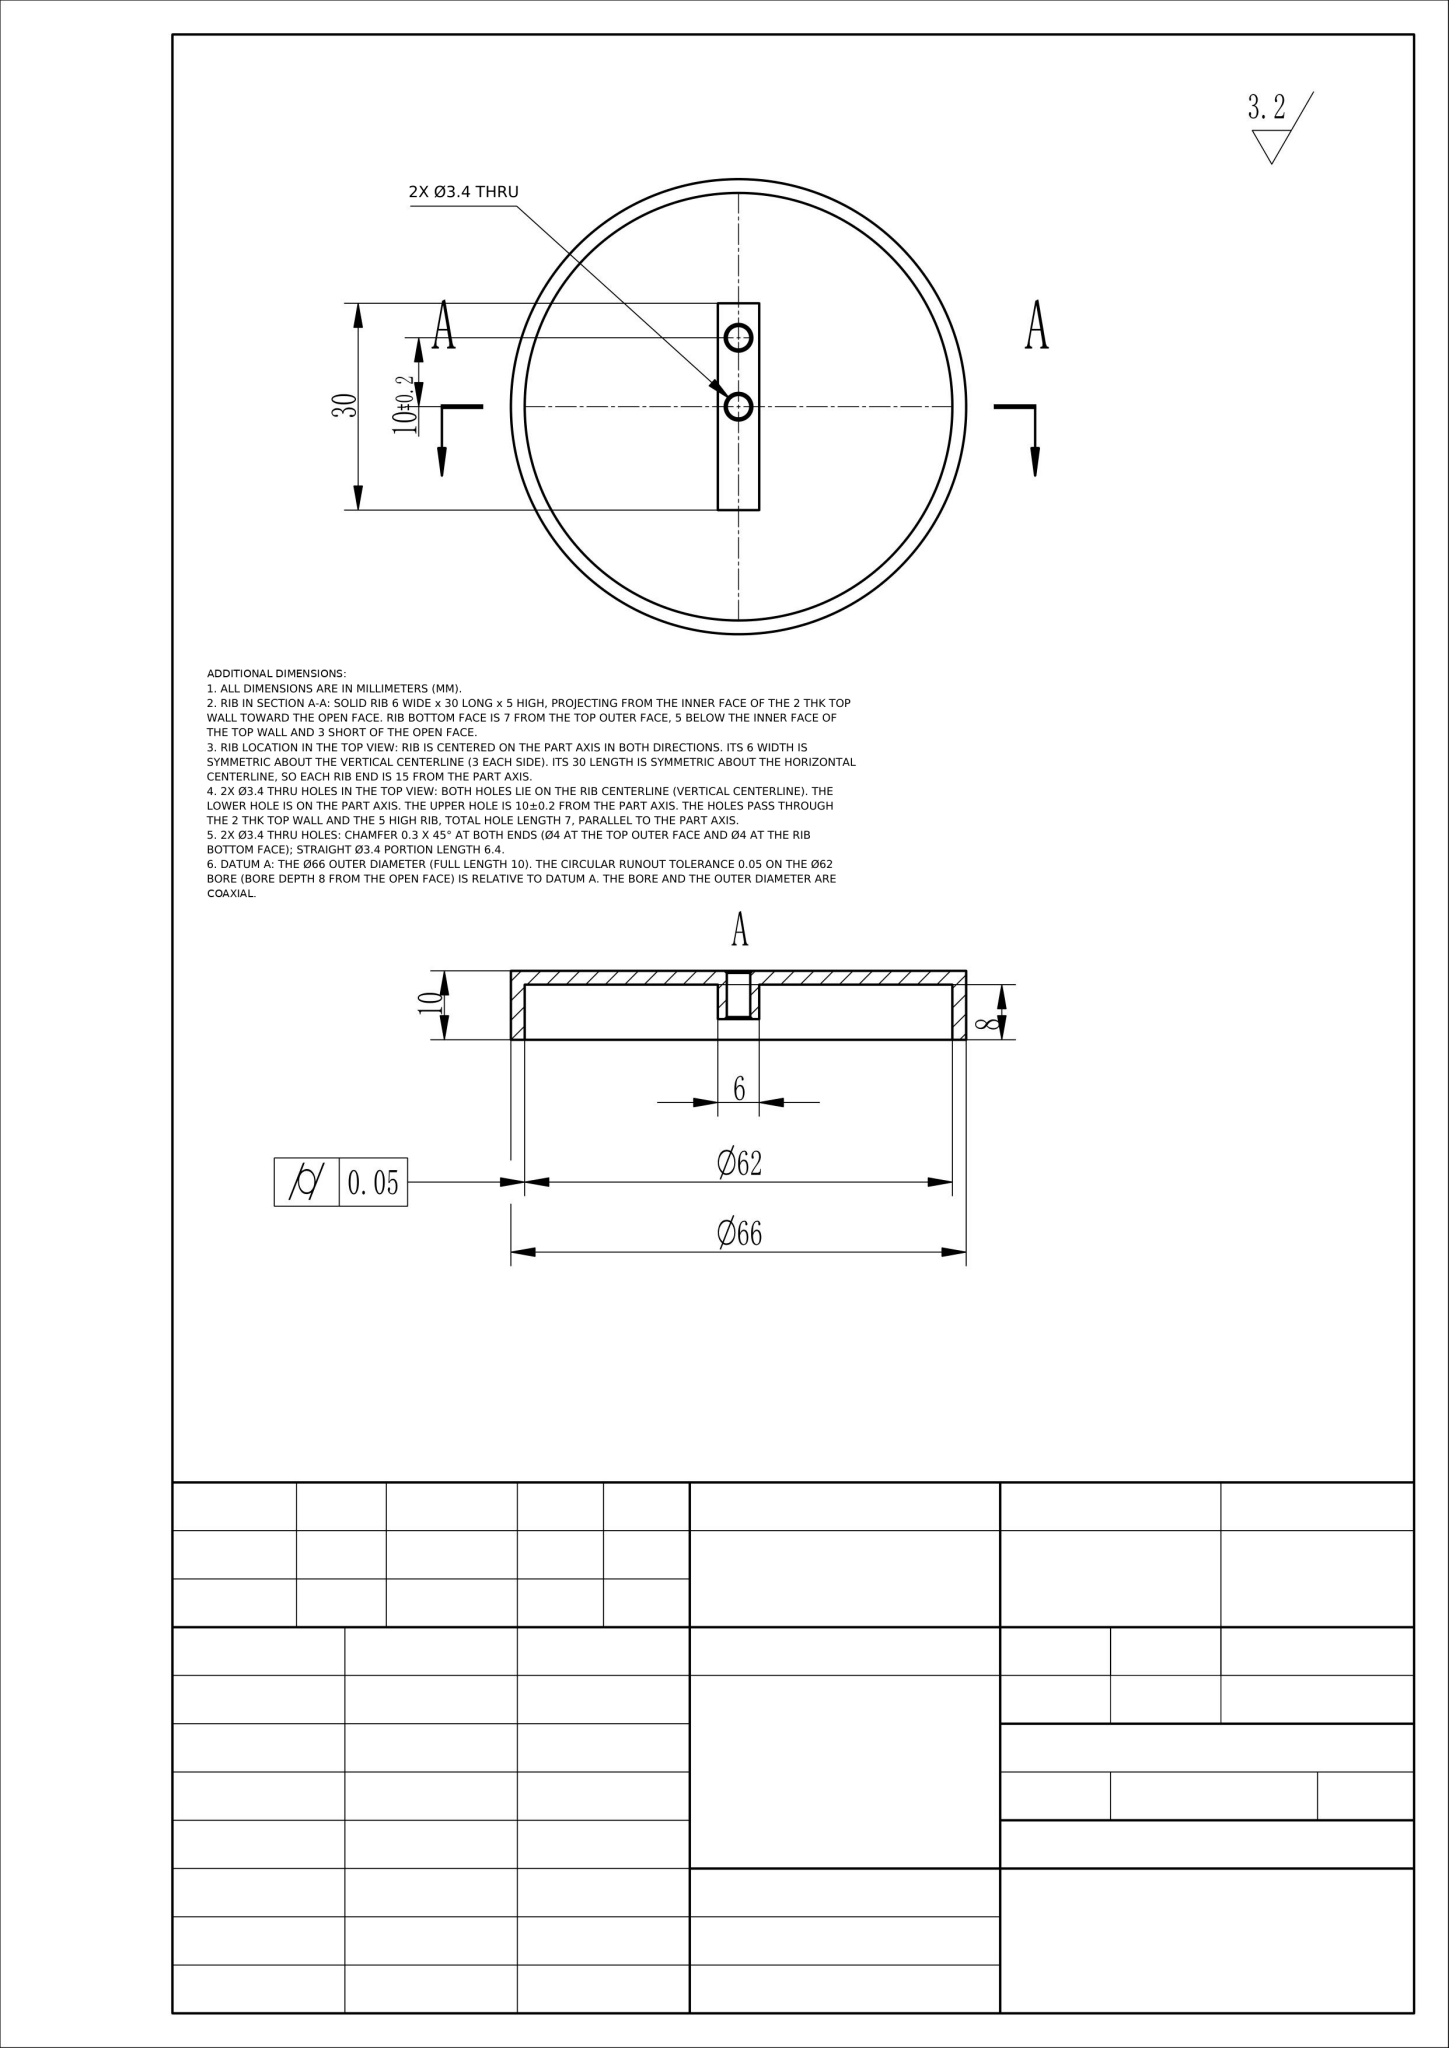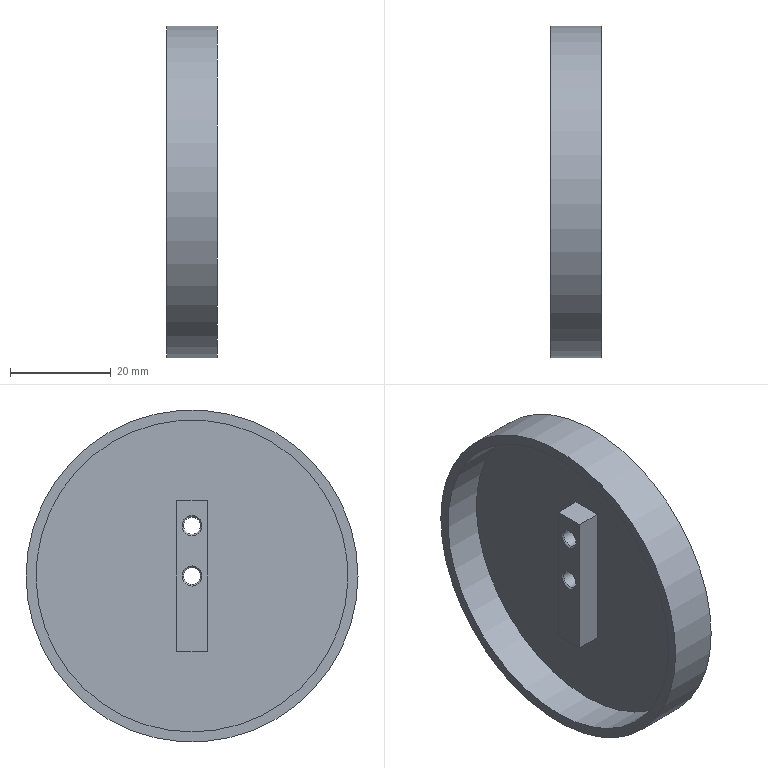Part | NX | mm | 1 solid | 16 faces | box 10 x 66 x 66 mm | volume 10830 mm3 | plane 8 | cylinder 4 | cone 4 | commonest cylinder face diameters 3.4 x2 62 x1 66 x1
STEP:
#1=CARTESIAN_POINT('',(0.,0.,0.));
#2=DIRECTION('',(0.,0.,1.));
#3=DIRECTION('',(1.,0.,0.));
#4=AXIS2_PLACEMENT_3D('',#1,#2,#3);
#5=(LENGTH_UNIT()NAMED_UNIT(*)SI_UNIT(.MILLI.,.METRE.));
#6=UNCERTAINTY_MEASURE_WITH_UNIT(LENGTH_MEASURE(0.00002),#5,'','');
#7=(NAMED_UNIT(*)PLANE_ANGLE_UNIT()SI_UNIT($,.RADIAN.));
#8=PLANE_ANGLE_MEASURE_WITH_UNIT(PLANE_ANGLE_MEASURE(0.01745),#7);
#9=DIMENSIONAL_EXPONENTS(0.,0.,0.,0.,0.,0.,0.);
#10=(CONVERSION_BASED_UNIT('',#8)NAMED_UNIT(#9)PLANE_ANGLE_UNIT());
#11=(NAMED_UNIT(*)SI_UNIT($,.STERADIAN.)SOLID_ANGLE_UNIT());
#12=(GEOMETRIC_REPRESENTATION_CONTEXT(3)GLOBAL_UNCERTAINTY_ASSIGNED_CONTEXT((#6))GLOBAL_UNIT_ASSIGNED_CONTEXT((#5,#10,#11))REPRESENTATION_CONTEXT('',''));
#13=SHAPE_REPRESENTATION('',(#4),#12);
#14=CARTESIAN_POINT('',(6.,0.,-31.));
#15=VERTEX_POINT('',#14);
#16=CARTESIAN_POINT('',(6.,0.,0.));
#17=DIRECTION('',(1.,0.,0.));
#18=DIRECTION('',(0.,0.,-1.));
#19=AXIS2_PLACEMENT_3D('',#16,#17,#18);
#20=CIRCLE('',#19,31.);
#21=EDGE_CURVE('',#15,#15,#20,.T.);
#22=ORIENTED_EDGE('',*,*,#21,.F.);
#23=EDGE_LOOP('',(#22));
#24=FACE_BOUND('',#23,.T.);
#25=CARTESIAN_POINT('',(6.,-3.,-15.));
#26=VERTEX_POINT('',#25);
#27=CARTESIAN_POINT('',(6.,-3.,15.));
#28=VERTEX_POINT('',#27);
#29=CARTESIAN_POINT('',(6.,-3.,-15.));
#30=DIRECTION('',(0.,0.,1.));
#31=VECTOR('',#30,1.);
#32=LINE('',#29,#31);
#33=EDGE_CURVE('',#26,#28,#32,.T.);
#34=ORIENTED_EDGE('',*,*,#33,.F.);
#35=CARTESIAN_POINT('',(6.,3.,-15.));
#36=VERTEX_POINT('',#35);
#37=CARTESIAN_POINT('',(6.,3.,-15.));
#38=DIRECTION('',(0.,-1.,0.));
#39=VECTOR('',#38,1.);
#40=LINE('',#37,#39);
#41=EDGE_CURVE('',#36,#26,#40,.T.);
#42=ORIENTED_EDGE('',*,*,#41,.F.);
#43=CARTESIAN_POINT('',(6.,3.,15.));
#44=VERTEX_POINT('',#43);
#45=CARTESIAN_POINT('',(6.,3.,15.));
#46=DIRECTION('',(0.,-0.,-1.));
#47=VECTOR('',#46,1.);
#48=LINE('',#45,#47);
#49=EDGE_CURVE('',#44,#36,#48,.T.);
#50=ORIENTED_EDGE('',*,*,#49,.F.);
#51=CARTESIAN_POINT('',(6.,-3.,15.));
#52=DIRECTION('',(0.,1.,0.));
#53=VECTOR('',#52,1.);
#54=LINE('',#51,#53);
#55=EDGE_CURVE('',#28,#44,#54,.T.);
#56=ORIENTED_EDGE('',*,*,#55,.F.);
#57=EDGE_LOOP('',(#34,#42,#50,#56));
#58=FACE_BOUND('',#57,.T.);
#59=CARTESIAN_POINT('',(6.,0.,0.));
#60=DIRECTION('',(1.,0.,0.));
#61=DIRECTION('',(0.,0.,-1.));
#62=AXIS2_PLACEMENT_3D('',#59,#60,#61);
#63=PLANE('',#62);
#64=ADVANCED_FACE('',(#24,#58),#63,.F.);
#65=CARTESIAN_POINT('',(-2.,0.,-31.));
#66=VERTEX_POINT('',#65);
#67=CARTESIAN_POINT('',(-2.,0.,0.));
#68=DIRECTION('',(1.,0.,0.));
#69=DIRECTION('',(0.,0.,-1.));
#70=AXIS2_PLACEMENT_3D('',#67,#68,#69);
#71=CIRCLE('',#70,31.);
#72=EDGE_CURVE('',#66,#66,#71,.T.);
#73=ORIENTED_EDGE('',*,*,#72,.F.);
#74=EDGE_LOOP('',(#73));
#75=FACE_BOUND('',#74,.T.);
#76=ORIENTED_EDGE('',*,*,#21,.T.);
#77=EDGE_LOOP('',(#76));
#78=FACE_BOUND('',#77,.T.);
#79=CARTESIAN_POINT('',(8.,0.,0.));
#80=DIRECTION('',(-1.,0.,0.));
#81=DIRECTION('',(0.,0.,1.));
#82=AXIS2_PLACEMENT_3D('',#79,#80,#81);
#83=CYLINDRICAL_SURFACE('',#82,31.);
#84=ADVANCED_FACE('',(#75,#78),#83,.F.);
#85=CARTESIAN_POINT('',(8.,33.,-0.));
#86=VERTEX_POINT('',#85);
#87=CARTESIAN_POINT('',(8.,0.,0.));
#88=DIRECTION('',(1.,0.,0.));
#89=DIRECTION('',(0.,1.,-0.));
#90=AXIS2_PLACEMENT_3D('',#87,#88,#89);
#91=CIRCLE('',#90,33.);
#92=EDGE_CURVE('',#86,#86,#91,.T.);
#93=ORIENTED_EDGE('',*,*,#92,.F.);
#94=EDGE_LOOP('',(#93));
#95=FACE_BOUND('',#94,.T.);
#96=CARTESIAN_POINT('',(-2.,33.,-0.));
#97=VERTEX_POINT('',#96);
#98=CARTESIAN_POINT('',(-2.,0.,0.));
#99=DIRECTION('',(1.,0.,0.));
#100=DIRECTION('',(0.,1.,-0.));
#101=AXIS2_PLACEMENT_3D('',#98,#99,#100);
#102=CIRCLE('',#101,33.);
#103=EDGE_CURVE('',#97,#97,#102,.T.);
#104=ORIENTED_EDGE('',*,*,#103,.T.);
#105=EDGE_LOOP('',(#104));
#106=FACE_BOUND('',#105,.T.);
#107=CARTESIAN_POINT('',(8.,0.,0.));
#108=DIRECTION('',(-1.,0.,0.));
#109=DIRECTION('',(0.,0.,1.));
#110=AXIS2_PLACEMENT_3D('',#107,#108,#109);
#111=CYLINDRICAL_SURFACE('',#110,33.);
#112=ADVANCED_FACE('',(#95,#106),#111,.T.);
#113=CARTESIAN_POINT('',(8.,-0.,-2.));
#114=VERTEX_POINT('',#113);
#115=CARTESIAN_POINT('',(8.,-0.,0.));
#116=DIRECTION('',(-1.,0.,0.));
#117=DIRECTION('',(0.,0.,-1.));
#118=AXIS2_PLACEMENT_3D('',#115,#116,#117);
#119=CIRCLE('',#118,2.);
#120=EDGE_CURVE('',#114,#114,#119,.T.);
#121=ORIENTED_EDGE('',*,*,#120,.T.);
#122=EDGE_LOOP('',(#121));
#123=FACE_BOUND('',#122,.T.);
#124=CARTESIAN_POINT('',(8.,0.,8.));
#125=VERTEX_POINT('',#124);
#126=CARTESIAN_POINT('',(8.,0.,10.));
#127=DIRECTION('',(-1.,0.,0.));
#128=DIRECTION('',(0.,0.,-1.));
#129=AXIS2_PLACEMENT_3D('',#126,#127,#128);
#130=CIRCLE('',#129,2.);
#131=EDGE_CURVE('',#125,#125,#130,.T.);
#132=ORIENTED_EDGE('',*,*,#131,.T.);
#133=EDGE_LOOP('',(#132));
#134=FACE_BOUND('',#133,.T.);
#135=ORIENTED_EDGE('',*,*,#92,.T.);
#136=EDGE_LOOP('',(#135));
#137=FACE_BOUND('',#136,.T.);
#138=CARTESIAN_POINT('',(8.,0.,0.));
#139=DIRECTION('',(1.,0.,0.));
#140=DIRECTION('',(0.,0.,-1.));
#141=AXIS2_PLACEMENT_3D('',#138,#139,#140);
#142=PLANE('',#141);
#143=ADVANCED_FACE('',(#123,#134,#137),#142,.T.);
#144=ORIENTED_EDGE('',*,*,#103,.F.);
#145=EDGE_LOOP('',(#144));
#146=FACE_BOUND('',#145,.T.);
#147=ORIENTED_EDGE('',*,*,#72,.T.);
#148=EDGE_LOOP('',(#147));
#149=FACE_BOUND('',#148,.T.);
#150=CARTESIAN_POINT('',(-2.,0.,0.));
#151=DIRECTION('',(1.,0.,0.));
#152=DIRECTION('',(0.,0.,-1.));
#153=AXIS2_PLACEMENT_3D('',#150,#151,#152);
#154=PLANE('',#153);
#155=ADVANCED_FACE('',(#146,#149),#154,.F.);
#156=ORIENTED_EDGE('',*,*,#33,.T.);
#157=CARTESIAN_POINT('',(1.,-3.,15.));
#158=VERTEX_POINT('',#157);
#159=CARTESIAN_POINT('',(1.,-3.,15.));
#160=DIRECTION('',(1.,0.,0.));
#161=VECTOR('',#160,1.);
#162=LINE('',#159,#161);
#163=EDGE_CURVE('',#158,#28,#162,.T.);
#164=ORIENTED_EDGE('',*,*,#163,.F.);
#165=CARTESIAN_POINT('',(1.,-3.,-15.));
#166=VERTEX_POINT('',#165);
#167=CARTESIAN_POINT('',(1.,-3.,-15.));
#168=DIRECTION('',(0.,0.,1.));
#169=VECTOR('',#168,1.);
#170=LINE('',#167,#169);
#171=EDGE_CURVE('',#166,#158,#170,.T.);
#172=ORIENTED_EDGE('',*,*,#171,.F.);
#173=CARTESIAN_POINT('',(1.,-3.,-15.));
#174=DIRECTION('',(1.,0.,0.));
#175=VECTOR('',#174,1.);
#176=LINE('',#173,#175);
#177=EDGE_CURVE('',#166,#26,#176,.T.);
#178=ORIENTED_EDGE('',*,*,#177,.T.);
#179=EDGE_LOOP('',(#156,#164,#172,#178));
#180=FACE_OUTER_BOUND('',#179,.T.);
#181=CARTESIAN_POINT('',(1.,-3.,-15.));
#182=DIRECTION('',(0.,1.,-0.));
#183=DIRECTION('',(0.,0.,1.));
#184=AXIS2_PLACEMENT_3D('',#181,#182,#183);
#185=PLANE('',#184);
#186=ADVANCED_FACE('',(#180),#185,.F.);
#187=ORIENTED_EDGE('',*,*,#55,.T.);
#188=CARTESIAN_POINT('',(1.,3.,15.));
#189=VERTEX_POINT('',#188);
#190=CARTESIAN_POINT('',(1.,3.,15.));
#191=DIRECTION('',(1.,0.,0.));
#192=VECTOR('',#191,1.);
#193=LINE('',#190,#192);
#194=EDGE_CURVE('',#189,#44,#193,.T.);
#195=ORIENTED_EDGE('',*,*,#194,.F.);
#196=CARTESIAN_POINT('',(1.,-3.,15.));
#197=DIRECTION('',(0.,1.,0.));
#198=VECTOR('',#197,1.);
#199=LINE('',#196,#198);
#200=EDGE_CURVE('',#158,#189,#199,.T.);
#201=ORIENTED_EDGE('',*,*,#200,.F.);
#202=ORIENTED_EDGE('',*,*,#163,.T.);
#203=EDGE_LOOP('',(#187,#195,#201,#202));
#204=FACE_OUTER_BOUND('',#203,.T.);
#205=CARTESIAN_POINT('',(1.,-3.,15.));
#206=DIRECTION('',(0.,0.,-1.));
#207=DIRECTION('',(-1.,0.,0.));
#208=AXIS2_PLACEMENT_3D('',#205,#206,#207);
#209=PLANE('',#208);
#210=ADVANCED_FACE('',(#204),#209,.F.);
#211=ORIENTED_EDGE('',*,*,#49,.T.);
#212=CARTESIAN_POINT('',(1.,3.,-15.));
#213=VERTEX_POINT('',#212);
#214=CARTESIAN_POINT('',(1.,3.,-15.));
#215=DIRECTION('',(1.,0.,0.));
#216=VECTOR('',#215,1.);
#217=LINE('',#214,#216);
#218=EDGE_CURVE('',#213,#36,#217,.T.);
#219=ORIENTED_EDGE('',*,*,#218,.F.);
#220=CARTESIAN_POINT('',(1.,3.,15.));
#221=DIRECTION('',(0.,-0.,-1.));
#222=VECTOR('',#221,1.);
#223=LINE('',#220,#222);
#224=EDGE_CURVE('',#189,#213,#223,.T.);
#225=ORIENTED_EDGE('',*,*,#224,.F.);
#226=ORIENTED_EDGE('',*,*,#194,.T.);
#227=EDGE_LOOP('',(#211,#219,#225,#226));
#228=FACE_OUTER_BOUND('',#227,.T.);
#229=CARTESIAN_POINT('',(1.,3.,15.));
#230=DIRECTION('',(0.,-1.,0.));
#231=DIRECTION('',(0.,-0.,-1.));
#232=AXIS2_PLACEMENT_3D('',#229,#230,#231);
#233=PLANE('',#232);
#234=ADVANCED_FACE('',(#228),#233,.F.);
#235=ORIENTED_EDGE('',*,*,#41,.T.);
#236=ORIENTED_EDGE('',*,*,#177,.F.);
#237=CARTESIAN_POINT('',(1.,3.,-15.));
#238=DIRECTION('',(0.,-1.,0.));
#239=VECTOR('',#238,1.);
#240=LINE('',#237,#239);
#241=EDGE_CURVE('',#213,#166,#240,.T.);
#242=ORIENTED_EDGE('',*,*,#241,.F.);
#243=ORIENTED_EDGE('',*,*,#218,.T.);
#244=EDGE_LOOP('',(#235,#236,#242,#243));
#245=FACE_OUTER_BOUND('',#244,.T.);
#246=CARTESIAN_POINT('',(1.,3.,-15.));
#247=DIRECTION('',(0.,0.,1.));
#248=DIRECTION('',(0.,-1.,0.));
#249=AXIS2_PLACEMENT_3D('',#246,#247,#248);
#250=PLANE('',#249);
#251=ADVANCED_FACE('',(#245),#250,.F.);
#252=CARTESIAN_POINT('',(1.,-0.,2.));
#253=VERTEX_POINT('',#252);
#254=CARTESIAN_POINT('',(1.,-0.,0.));
#255=DIRECTION('',(1.,0.,0.));
#256=DIRECTION('',(0.,0.,1.));
#257=AXIS2_PLACEMENT_3D('',#254,#255,#256);
#258=CIRCLE('',#257,2.);
#259=EDGE_CURVE('',#253,#253,#258,.T.);
#260=ORIENTED_EDGE('',*,*,#259,.T.);
#261=EDGE_LOOP('',(#260));
#262=FACE_BOUND('',#261,.T.);
#263=CARTESIAN_POINT('',(1.,0.,12.));
#264=VERTEX_POINT('',#263);
#265=CARTESIAN_POINT('',(1.,0.,10.));
#266=DIRECTION('',(1.,0.,0.));
#267=DIRECTION('',(0.,0.,1.));
#268=AXIS2_PLACEMENT_3D('',#265,#266,#267);
#269=CIRCLE('',#268,2.);
#270=EDGE_CURVE('',#264,#264,#269,.T.);
#271=ORIENTED_EDGE('',*,*,#270,.T.);
#272=EDGE_LOOP('',(#271));
#273=FACE_BOUND('',#272,.T.);
#274=ORIENTED_EDGE('',*,*,#171,.T.);
#275=ORIENTED_EDGE('',*,*,#200,.T.);
#276=ORIENTED_EDGE('',*,*,#224,.T.);
#277=ORIENTED_EDGE('',*,*,#241,.T.);
#278=EDGE_LOOP('',(#274,#275,#276,#277));
#279=FACE_BOUND('',#278,.T.);
#280=CARTESIAN_POINT('',(1.,0.,0.));
#281=DIRECTION('',(-1.,0.,0.));
#282=DIRECTION('',(0.,0.,1.));
#283=AXIS2_PLACEMENT_3D('',#280,#281,#282);
#284=PLANE('',#283);
#285=ADVANCED_FACE('',(#262,#273,#279),#284,.T.);
#286=CARTESIAN_POINT('',(7.7,0.,8.3));
#287=VERTEX_POINT('',#286);
#288=CARTESIAN_POINT('',(7.7,0.,10.));
#289=DIRECTION('',(1.,0.,0.));
#290=DIRECTION('',(0.,0.,-1.));
#291=AXIS2_PLACEMENT_3D('',#288,#289,#290);
#292=CIRCLE('',#291,1.7);
#293=EDGE_CURVE('',#287,#287,#292,.T.);
#294=ORIENTED_EDGE('',*,*,#293,.T.);
#295=EDGE_LOOP('',(#294));
#296=FACE_BOUND('',#295,.T.);
#297=CARTESIAN_POINT('',(1.3,0.,11.7));
#298=VERTEX_POINT('',#297);
#299=CARTESIAN_POINT('',(1.3,0.,10.));
#300=DIRECTION('',(-1.,0.,0.));
#301=DIRECTION('',(0.,0.,1.));
#302=AXIS2_PLACEMENT_3D('',#299,#300,#301);
#303=CIRCLE('',#302,1.7);
#304=EDGE_CURVE('',#298,#298,#303,.T.);
#305=ORIENTED_EDGE('',*,*,#304,.T.);
#306=EDGE_LOOP('',(#305));
#307=FACE_BOUND('',#306,.T.);
#308=CARTESIAN_POINT('',(1.,0.,10.));
#309=DIRECTION('',(1.,0.,0.));
#310=DIRECTION('',(0.,0.,-1.));
#311=AXIS2_PLACEMENT_3D('',#308,#309,#310);
#312=CYLINDRICAL_SURFACE('',#311,1.7);
#313=ADVANCED_FACE('',(#296,#307),#312,.F.);
#314=ORIENTED_EDGE('',*,*,#304,.F.);
#315=EDGE_LOOP('',(#314));
#316=FACE_BOUND('',#315,.T.);
#317=ORIENTED_EDGE('',*,*,#270,.F.);
#318=EDGE_LOOP('',(#317));
#319=FACE_BOUND('',#318,.T.);
#320=CARTESIAN_POINT('',(1.,0.,10.));
#321=DIRECTION('',(-1.,0.,0.));
#322=DIRECTION('',(0.,0.,1.));
#323=AXIS2_PLACEMENT_3D('',#320,#321,#322);
#324=CONICAL_SURFACE('',#323,2.,45.);
#325=ADVANCED_FACE('',(#316,#319),#324,.F.);
#326=ORIENTED_EDGE('',*,*,#131,.F.);
#327=EDGE_LOOP('',(#326));
#328=FACE_BOUND('',#327,.T.);
#329=ORIENTED_EDGE('',*,*,#293,.F.);
#330=EDGE_LOOP('',(#329));
#331=FACE_BOUND('',#330,.T.);
#332=CARTESIAN_POINT('',(7.7,0.,10.));
#333=DIRECTION('',(1.,0.,0.));
#334=DIRECTION('',(0.,0.,-1.));
#335=AXIS2_PLACEMENT_3D('',#332,#333,#334);
#336=CONICAL_SURFACE('',#335,1.7,45.);
#337=ADVANCED_FACE('',(#328,#331),#336,.F.);
#338=CARTESIAN_POINT('',(7.7,-0.,-1.7));
#339=VERTEX_POINT('',#338);
#340=CARTESIAN_POINT('',(7.7,-0.,0.));
#341=DIRECTION('',(1.,0.,0.));
#342=DIRECTION('',(0.,0.,-1.));
#343=AXIS2_PLACEMENT_3D('',#340,#341,#342);
#344=CIRCLE('',#343,1.7);
#345=EDGE_CURVE('',#339,#339,#344,.T.);
#346=ORIENTED_EDGE('',*,*,#345,.T.);
#347=EDGE_LOOP('',(#346));
#348=FACE_BOUND('',#347,.T.);
#349=CARTESIAN_POINT('',(1.3,-0.,1.7));
#350=VERTEX_POINT('',#349);
#351=CARTESIAN_POINT('',(1.3,-0.,0.));
#352=DIRECTION('',(-1.,0.,0.));
#353=DIRECTION('',(0.,0.,1.));
#354=AXIS2_PLACEMENT_3D('',#351,#352,#353);
#355=CIRCLE('',#354,1.7);
#356=EDGE_CURVE('',#350,#350,#355,.T.);
#357=ORIENTED_EDGE('',*,*,#356,.T.);
#358=EDGE_LOOP('',(#357));
#359=FACE_BOUND('',#358,.T.);
#360=CARTESIAN_POINT('',(1.,-0.,0.));
#361=DIRECTION('',(1.,0.,0.));
#362=DIRECTION('',(0.,0.,-1.));
#363=AXIS2_PLACEMENT_3D('',#360,#361,#362);
#364=CYLINDRICAL_SURFACE('',#363,1.7);
#365=ADVANCED_FACE('',(#348,#359),#364,.F.);
#366=ORIENTED_EDGE('',*,*,#356,.F.);
#367=EDGE_LOOP('',(#366));
#368=FACE_BOUND('',#367,.T.);
#369=ORIENTED_EDGE('',*,*,#259,.F.);
#370=EDGE_LOOP('',(#369));
#371=FACE_BOUND('',#370,.T.);
#372=CARTESIAN_POINT('',(1.,-0.,0.));
#373=DIRECTION('',(-1.,0.,0.));
#374=DIRECTION('',(0.,0.,1.));
#375=AXIS2_PLACEMENT_3D('',#372,#373,#374);
#376=CONICAL_SURFACE('',#375,2.,45.);
#377=ADVANCED_FACE('',(#368,#371),#376,.F.);
#378=ORIENTED_EDGE('',*,*,#120,.F.);
#379=EDGE_LOOP('',(#378));
#380=FACE_BOUND('',#379,.T.);
#381=ORIENTED_EDGE('',*,*,#345,.F.);
#382=EDGE_LOOP('',(#381));
#383=FACE_BOUND('',#382,.T.);
#384=CARTESIAN_POINT('',(7.7,-0.,0.));
#385=DIRECTION('',(1.,0.,0.));
#386=DIRECTION('',(0.,0.,-1.));
#387=AXIS2_PLACEMENT_3D('',#384,#385,#386);
#388=CONICAL_SURFACE('',#387,1.7,45.);
#389=ADVANCED_FACE('',(#380,#383),#388,.F.);
#390=CLOSED_SHELL('',(#64,#84,#112,#143,#155,#186,#210,#234,#251,#285,#313,#325,#337,#365,#377,#389));
#391=MANIFOLD_SOLID_BREP('',#390);
#392=ADVANCED_BREP_SHAPE_REPRESENTATION('',(#391),#12);
#393=SHAPE_REPRESENTATION_RELATIONSHIP('','',#13,#392);
#394=PRESENTATION_LAYER_ASSIGNMENT('','',(#391));
#395=COLOUR_RGB('',1.,0.6,0.);
#396=FILL_AREA_STYLE_COLOUR('',#395);
#397=FILL_AREA_STYLE('',(#396));
#398=SURFACE_STYLE_FILL_AREA(#397);
#399=SURFACE_SIDE_STYLE('',(#398));
#400=SURFACE_STYLE_USAGE(.BOTH.,#399);
#401=PRESENTATION_STYLE_ASSIGNMENT((#400));
#402=STYLED_ITEM('',(#401),#391);
#403=MECHANICAL_DESIGN_GEOMETRIC_PRESENTATION_REPRESENTATION('',(#402),#12);